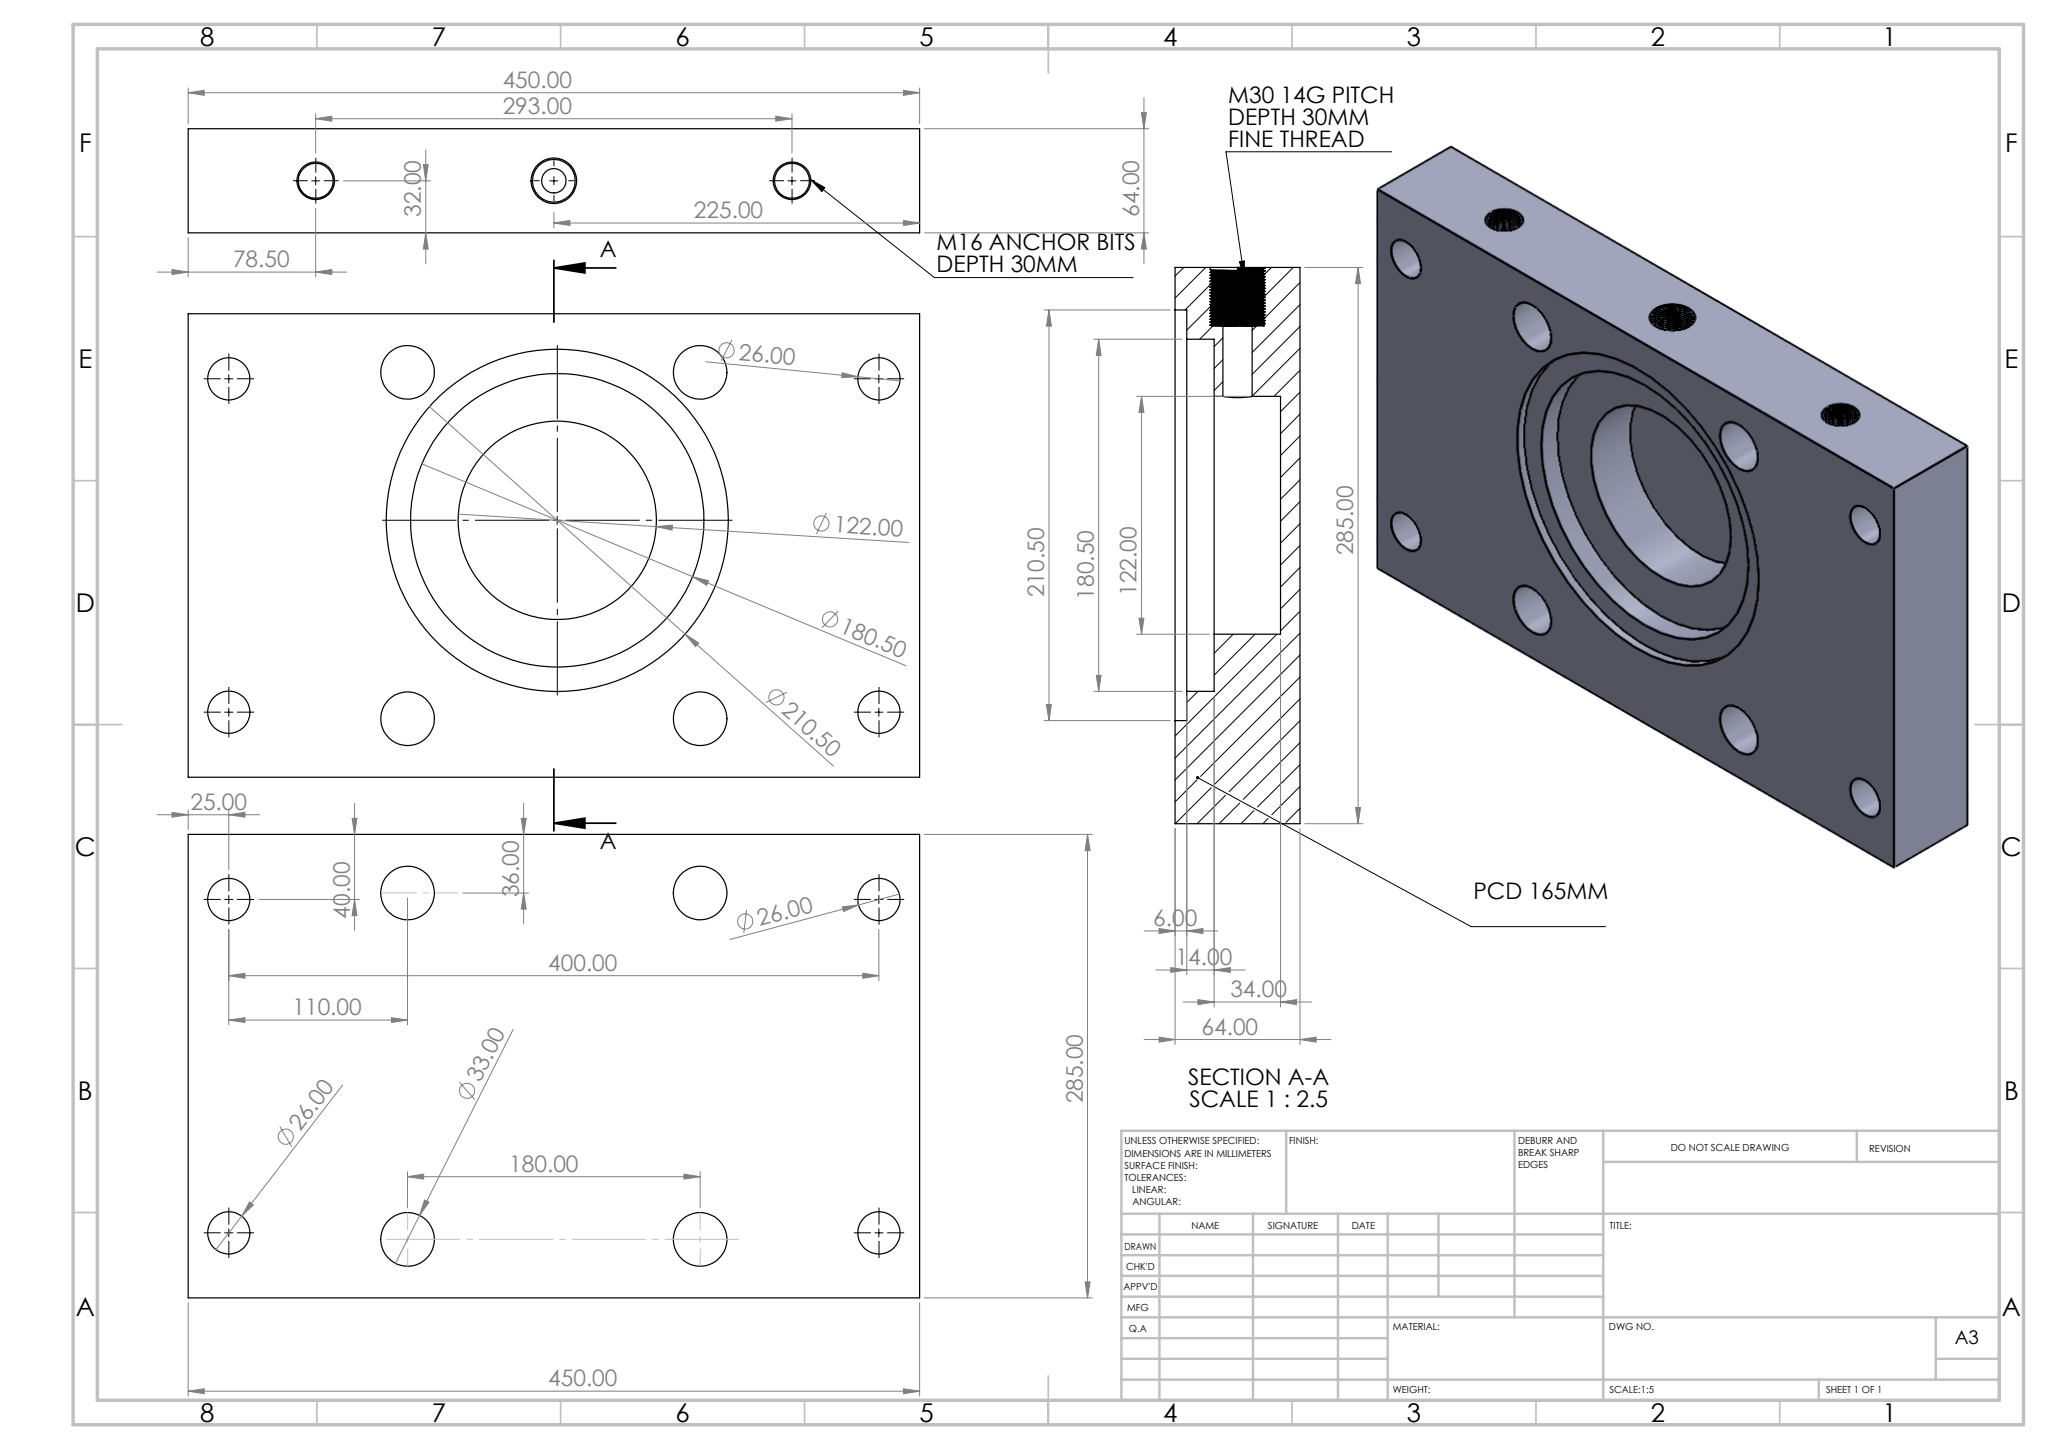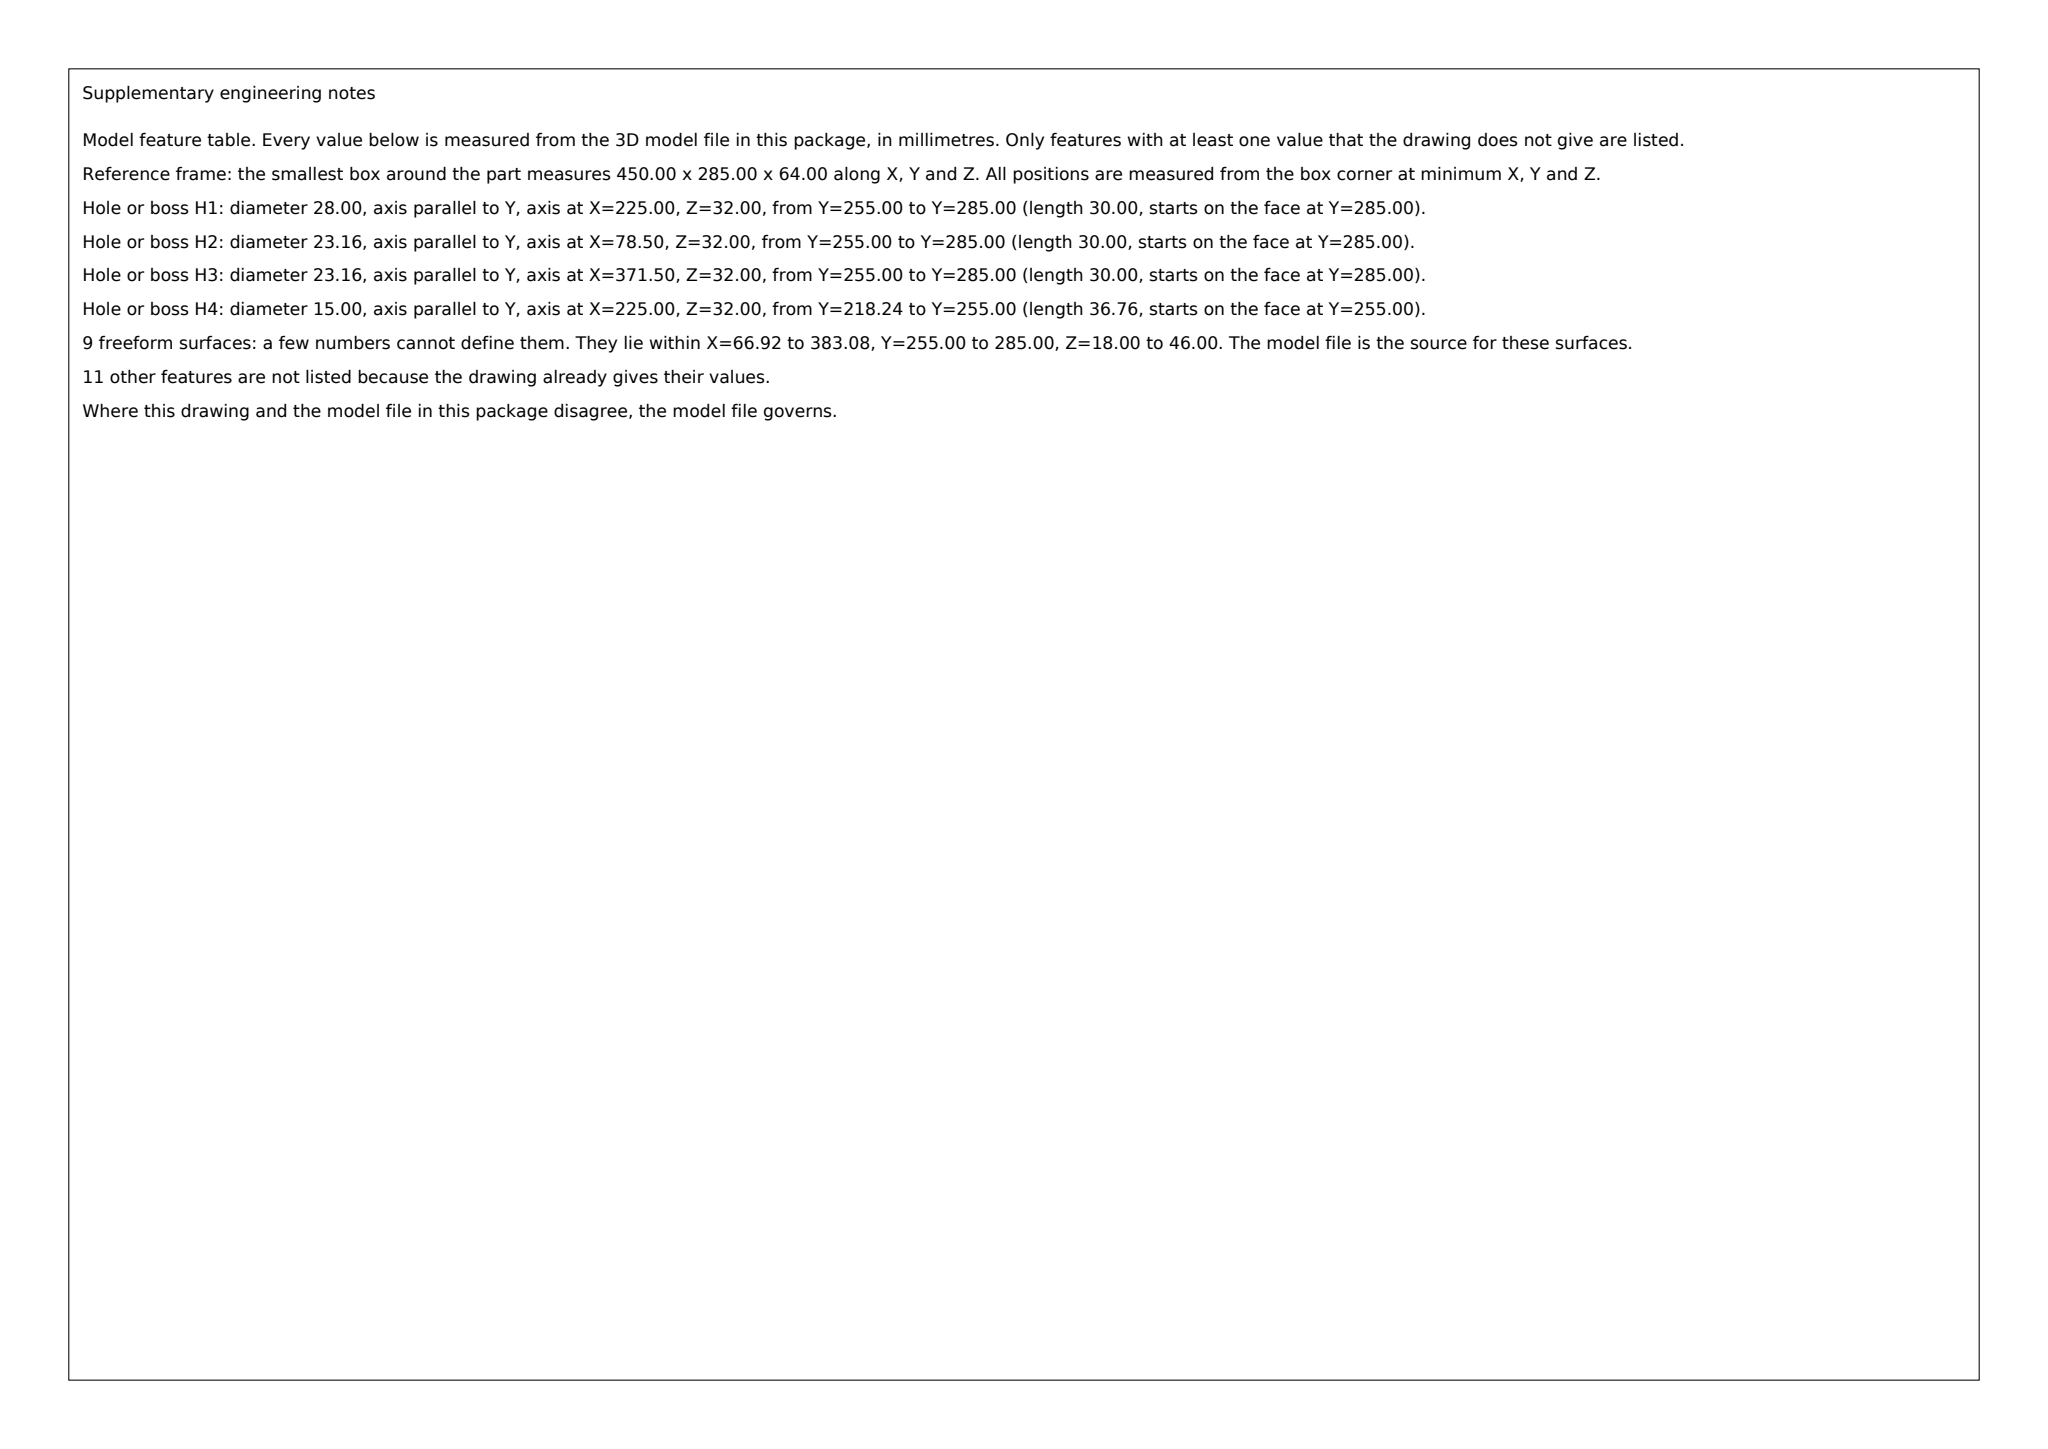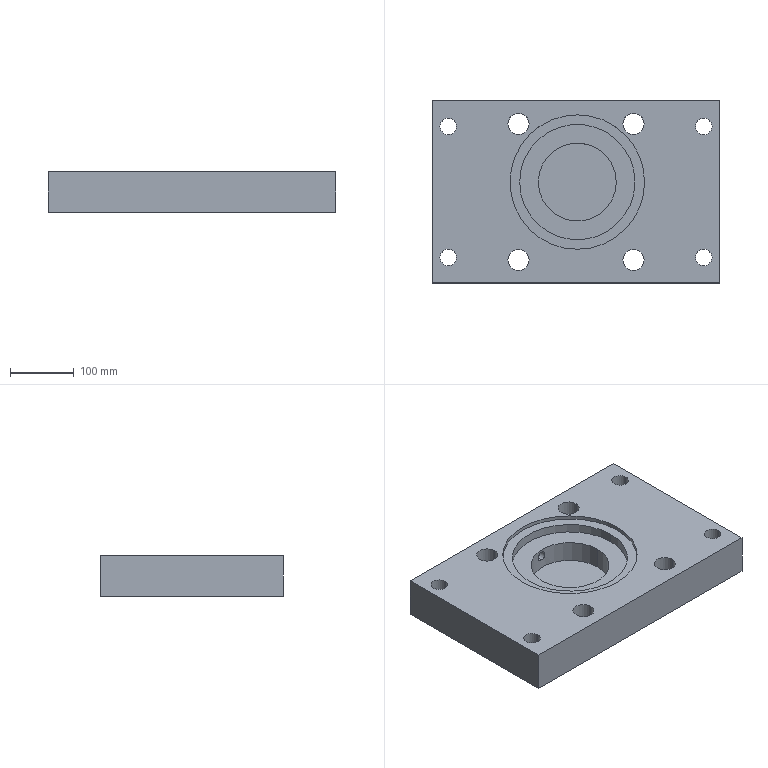Part | SolidWorks | mm | 1 solid | 171 faces | box 450 x 285 x 64 mm | volume 6841515 mm3 | cylinder 147 | plane 15 | spline 9 | commonest cylinder face diameters 23.16 x82 28 x41 33 x8 26 x8 15 x2 122 x2 180.5 x2 210.5 x2
Drawing notes:
Ø15 DRILL UNDER M30 TAP, DP 36 BELOW TAP INTO Ø122 BORE | from the solid: cyl dia 15, axis y at x=225, z=32, len 36.24/36.76 from y=255 (tap bottom) to bore face y≈218.5
UPPER ROW: Ø26 40 & Ø33 36 FROM TOP EDGE; SYM ABOUT HORIZ CL | from the solid: Ø26 at y=245, Ø33 at y=249; bbox y=285 so 40 and 36 from top, matching 40/36 at bottom
BORE AXIS: 227.09 FROM LH EDGE, 158 FROM BOTTOM EDGE | from the solid: Ø122/Ø180.5/Ø210.5 cyls all at pos (x=227.09, y=158), bbox 450x285
DELETE 'PCD 165MM': NO 165 BOLT CIRCLE ON PART | from the solid: no holes lie on any 165 dia circle; hole axes at x=25/135/315/425, y=36/40/245/249
2X M16 DP 30 ANCHOR, 1X M30 DP 30, 4X Ø26 THRU, 4X Ø33 THRU | from the solid: Ø23.16 thread cyls at x=78.5 & 371.5 (2), Ø28 at x=225 (1), Ø26 x4, Ø33 x4, len 64 = full thk